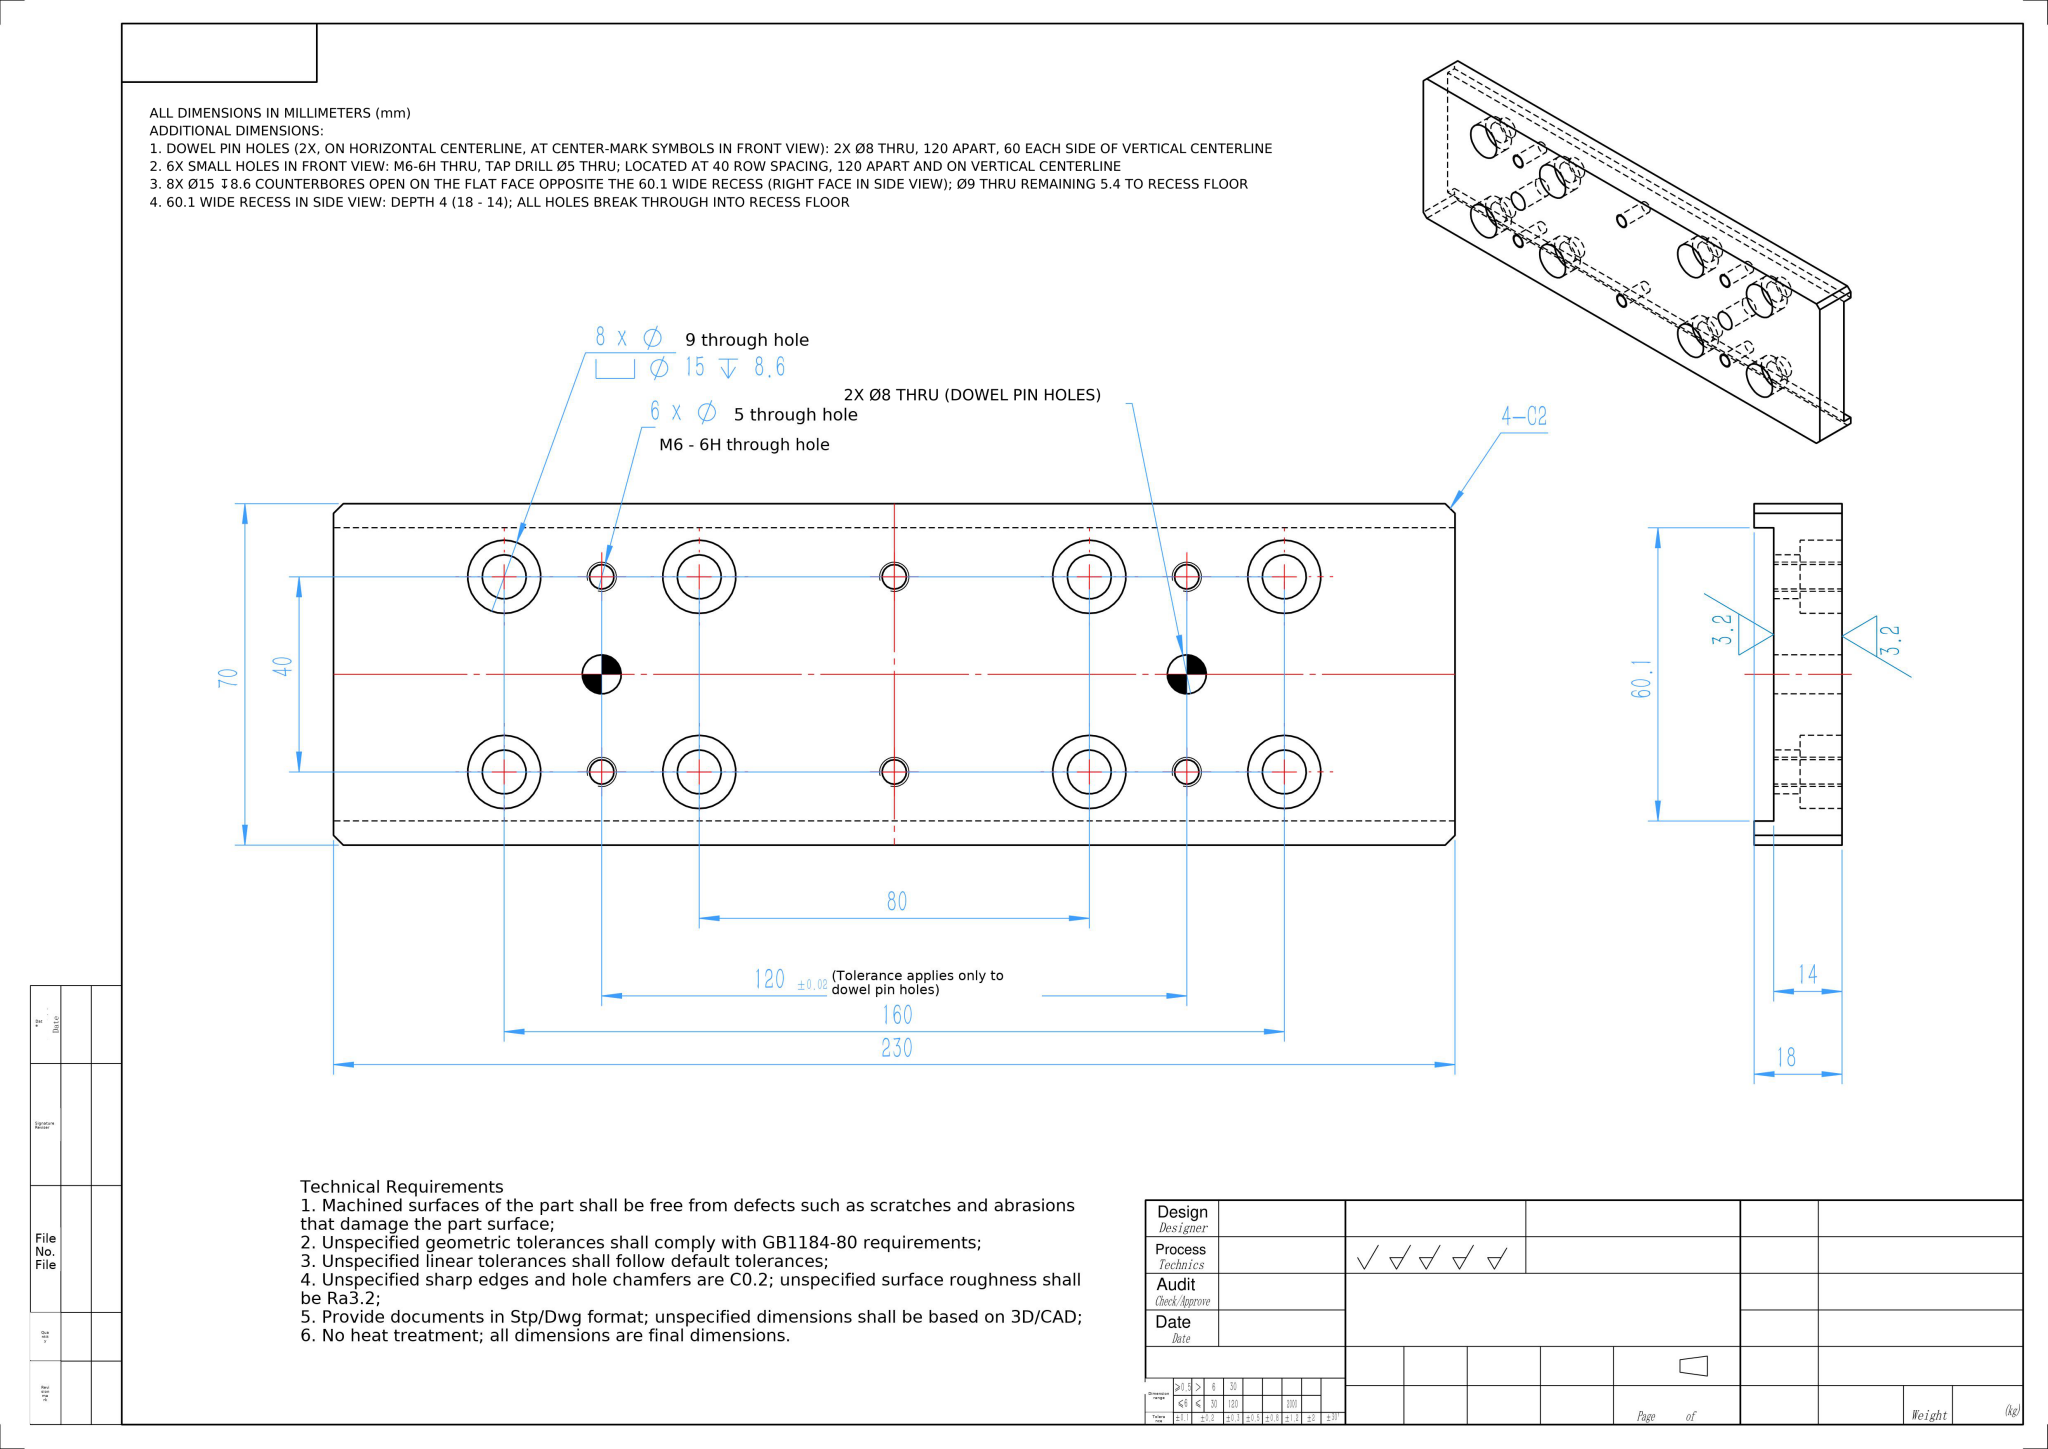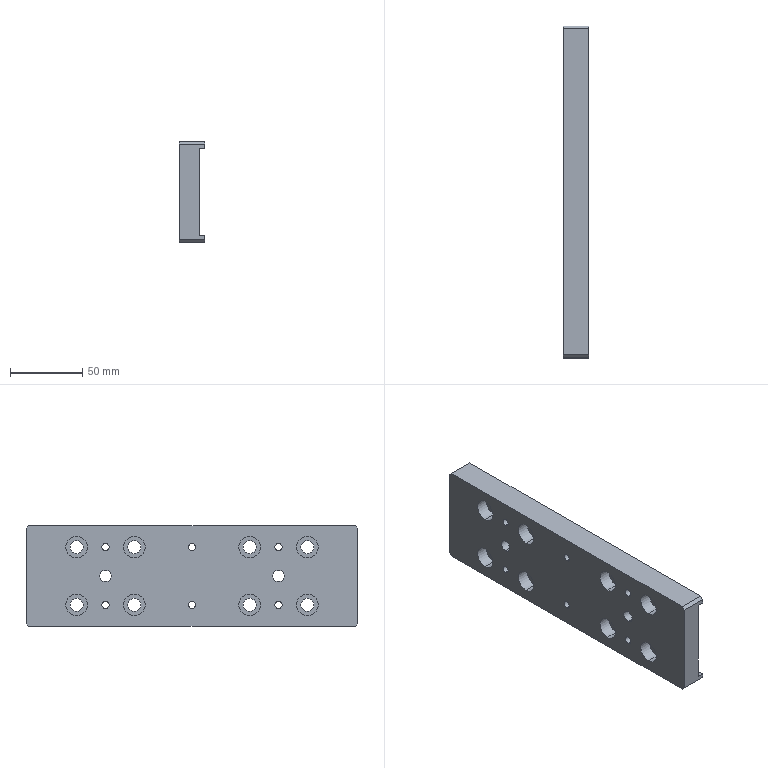Part | NX | mm | 1 solid | 70 faces | box 18 x 230 x 70 mm | volume 216401 mm3 | cylinder 48 | plane 22 | commonest cylinder face diameters 15 x16 9 x16 5 x12 8 x4